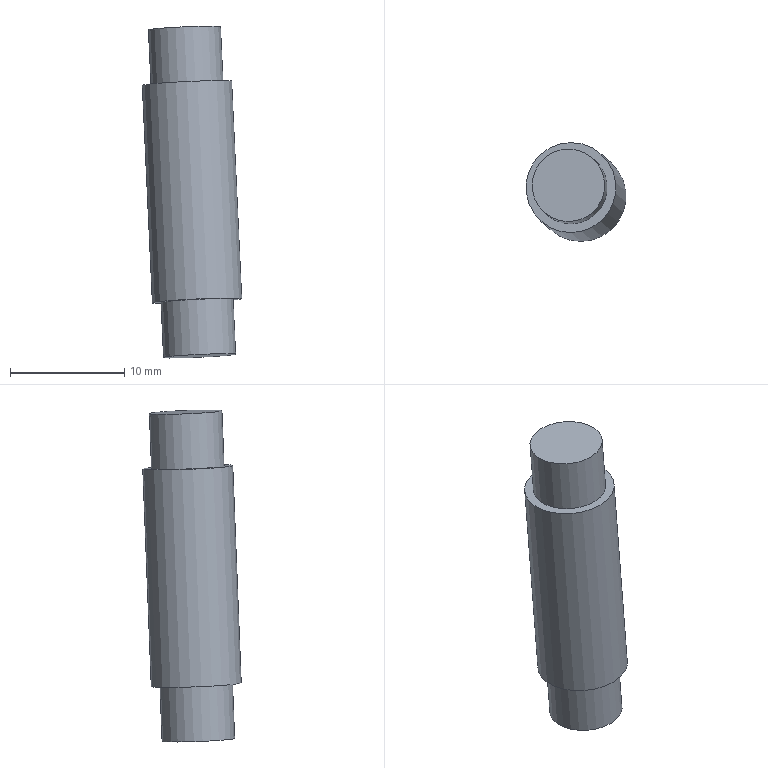Component | NX | PASADOR_A_2 | 1 solid | 7 faces | box 8.75 x 8.61 x 29.03 mm | volume 1233 mm3 | plane 4 | cylinder 3 | commonest cylinder face diameters 6.35 x2 7.874 x1
STEP:
#1=CARTESIAN_POINT('',(0.,0.,0.));
#2=DIRECTION('',(0.,0.,1.));
#3=DIRECTION('',(1.,0.,0.));
#4=AXIS2_PLACEMENT_3D('',#1,#2,#3);
#5=CARTESIAN_POINT('',(4.095,61.023,10.643));
#6=VERTEX_POINT('',#5);
#7=CARTESIAN_POINT('',(0.1942,61.516,10.443));
#8=DIRECTION('',(-0.04625,0.03881,0.9982));
#9=DIRECTION('',(0.9908,-0.1251,0.05077));
#10=AXIS2_PLACEMENT_3D('',#7,#8,#9);
#11=CIRCLE('',#10,3.937);
#12=CARTESIAN_POINT('',(0.1942,61.516,10.443));
#13=DIRECTION('',(-0.04625,0.03881,0.9982));
#14=DIRECTION('',(0.9908,-0.1251,0.05077));
#15=AXIS2_PLACEMENT_3D('',#12,#13,#14);
#16=PLANE('',#15);
#17=CARTESIAN_POINT('',(0.,0.));
#18=DIRECTION('',(1.,-0.));
#19=AXIS2_PLACEMENT_2D('',#17,#18);
#20=CIRCLE('',#19,3.937);
#21=(GEOMETRIC_REPRESENTATION_CONTEXT(2)PARAMETRIC_REPRESENTATION_CONTEXT()REPRESENTATION_CONTEXT('',''));
#22=DEFINITIONAL_REPRESENTATION('',(#20),#21);
#23=PCURVE('',#16,#22);
#24=CARTESIAN_POINT('',(0.1942,61.516,10.443));
#25=DIRECTION('',(0.04625,-0.03881,-0.9982));
#26=DIRECTION('',(-0.9908,0.1251,-0.05077));
#27=AXIS2_PLACEMENT_3D('',#24,#25,#26);
#28=CYLINDRICAL_SURFACE('',#27,3.937);
#29=CARTESIAN_POINT('',(9.425,0.));
#30=DIRECTION('',(-1.,0.));
#31=VECTOR('',#30,1.);
#32=LINE('',#29,#31);
#33=(GEOMETRIC_REPRESENTATION_CONTEXT(2)PARAMETRIC_REPRESENTATION_CONTEXT()REPRESENTATION_CONTEXT('',''));
#34=DEFINITIONAL_REPRESENTATION('',(#32),#33);
#35=PCURVE('',#28,#34);
#36=SURFACE_CURVE('',#11,(#23,#35),.PCURVE_S1.);
#37=EDGE_CURVE('',#6,#6,#36,.T.);
#38=ORIENTED_EDGE('',*,*,#37,.T.);
#39=EDGE_LOOP('',(#38));
#40=FACE_BOUND('',#39,.T.);
#41=CARTESIAN_POINT('',(3.34,61.119,10.604));
#42=VERTEX_POINT('',#41);
#43=CARTESIAN_POINT('',(0.1942,61.516,10.443));
#44=DIRECTION('',(0.04625,-0.03881,-0.9982));
#45=DIRECTION('',(0.9908,-0.1251,0.05077));
#46=AXIS2_PLACEMENT_3D('',#43,#44,#45);
#47=CIRCLE('',#46,3.175);
#48=CARTESIAN_POINT('',(3.175,-0.));
#49=CARTESIAN_POINT('',(3.175,-5.499));
#50=CARTESIAN_POINT('',(-1.587,-2.75));
#51=CARTESIAN_POINT('',(-6.35,0.));
#52=CARTESIAN_POINT('',(-1.587,2.75));
#53=CARTESIAN_POINT('',(3.175,5.499));
#54=CARTESIAN_POINT('',(3.175,-0.));
#55=(BOUNDED_CURVE()B_SPLINE_CURVE(2,(#48,#49,#50,#51,#52,#53,#54),.UNSPECIFIED.,.T.,.F.)B_SPLINE_CURVE_WITH_KNOTS((1,2,2,2,2,1),(-2.094,0.,2.094,4.189,6.283,8.378),.UNSPECIFIED.)CURVE()GEOMETRIC_REPRESENTATION_ITEM()RATIONAL_B_SPLINE_CURVE((1.,0.5,1.,0.5,1.,0.5,1.))REPRESENTATION_ITEM(''));
#56=(GEOMETRIC_REPRESENTATION_CONTEXT(2)PARAMETRIC_REPRESENTATION_CONTEXT()REPRESENTATION_CONTEXT('',''));
#57=DEFINITIONAL_REPRESENTATION('',(#55),#56);
#58=PCURVE('',#16,#57);
#59=CARTESIAN_POINT('',(-0.02899,61.703,15.26));
#60=DIRECTION('',(0.04625,-0.03881,-0.9982));
#61=DIRECTION('',(-0.9908,0.1251,-0.05077));
#62=AXIS2_PLACEMENT_3D('',#59,#60,#61);
#63=CYLINDRICAL_SURFACE('',#62,3.175);
#64=CARTESIAN_POINT('',(3.142,4.826));
#65=DIRECTION('',(1.,0.));
#66=VECTOR('',#65,1.);
#67=LINE('',#64,#66);
#68=(GEOMETRIC_REPRESENTATION_CONTEXT(2)PARAMETRIC_REPRESENTATION_CONTEXT()REPRESENTATION_CONTEXT('',''));
#69=DEFINITIONAL_REPRESENTATION('',(#67),#68);
#70=PCURVE('',#63,#69);
#71=SURFACE_CURVE('',#47,(#58,#70),.PCURVE_S1.);
#72=EDGE_CURVE('',#42,#42,#71,.T.);
#73=ORIENTED_EDGE('',*,*,#72,.T.);
#74=EDGE_LOOP('',(#73));
#75=FACE_BOUND('',#74,.T.);
#76=ADVANCED_FACE('',(#40,#75),#16,.T.);
#77=CARTESIAN_POINT('',(4.976,60.284,-8.372));
#78=VERTEX_POINT('',#77);
#79=CARTESIAN_POINT('',(1.075,60.777,-8.572));
#80=DIRECTION('',(-0.04625,0.03881,0.9982));
#81=DIRECTION('',(0.9908,-0.1251,0.05077));
#82=AXIS2_PLACEMENT_3D('',#79,#80,#81);
#83=CIRCLE('',#82,3.937);
#84=CARTESIAN_POINT('',(1.075,60.777,-8.572));
#85=DIRECTION('',(-0.04625,0.03881,0.9982));
#86=DIRECTION('',(0.9908,-0.1251,0.05077));
#87=AXIS2_PLACEMENT_3D('',#84,#85,#86);
#88=PLANE('',#87);
#89=CARTESIAN_POINT('',(0.,0.));
#90=DIRECTION('',(1.,-0.));
#91=AXIS2_PLACEMENT_2D('',#89,#90);
#92=CIRCLE('',#91,3.937);
#93=(GEOMETRIC_REPRESENTATION_CONTEXT(2)PARAMETRIC_REPRESENTATION_CONTEXT()REPRESENTATION_CONTEXT('',''));
#94=DEFINITIONAL_REPRESENTATION('',(#92),#93);
#95=PCURVE('',#88,#94);
#96=CARTESIAN_POINT('',(9.425,19.05));
#97=DIRECTION('',(-1.,0.));
#98=VECTOR('',#97,1.);
#99=LINE('',#96,#98);
#100=(GEOMETRIC_REPRESENTATION_CONTEXT(2)PARAMETRIC_REPRESENTATION_CONTEXT()REPRESENTATION_CONTEXT('',''));
#101=DEFINITIONAL_REPRESENTATION('',(#99),#100);
#102=PCURVE('',#28,#101);
#103=SURFACE_CURVE('',#83,(#95,#102),.PCURVE_S1.);
#104=EDGE_CURVE('',#78,#78,#103,.T.);
#105=ORIENTED_EDGE('',*,*,#104,.F.);
#106=EDGE_LOOP('',(#105));
#107=FACE_BOUND('',#106,.T.);
#108=CARTESIAN_POINT('',(4.221,60.38,-8.411));
#109=VERTEX_POINT('',#108);
#110=CARTESIAN_POINT('',(1.075,60.777,-8.572));
#111=DIRECTION('',(0.04625,-0.03881,-0.9982));
#112=DIRECTION('',(0.9908,-0.1251,0.05077));
#113=AXIS2_PLACEMENT_3D('',#110,#111,#112);
#114=CIRCLE('',#113,3.175);
#115=CARTESIAN_POINT('',(3.175,-0.));
#116=CARTESIAN_POINT('',(3.175,-5.499));
#117=CARTESIAN_POINT('',(-1.587,-2.75));
#118=CARTESIAN_POINT('',(-6.35,0.));
#119=CARTESIAN_POINT('',(-1.587,2.75));
#120=CARTESIAN_POINT('',(3.175,5.499));
#121=CARTESIAN_POINT('',(3.175,-0.));
#122=(BOUNDED_CURVE()B_SPLINE_CURVE(2,(#115,#116,#117,#118,#119,#120,#121),.UNSPECIFIED.,.T.,.F.)B_SPLINE_CURVE_WITH_KNOTS((1,2,2,2,2,1),(-2.094,0.,2.094,4.189,6.283,8.378),.UNSPECIFIED.)CURVE()GEOMETRIC_REPRESENTATION_ITEM()RATIONAL_B_SPLINE_CURVE((1.,0.5,1.,0.5,1.,0.5,1.))REPRESENTATION_ITEM(''));
#123=(GEOMETRIC_REPRESENTATION_CONTEXT(2)PARAMETRIC_REPRESENTATION_CONTEXT()REPRESENTATION_CONTEXT('',''));
#124=DEFINITIONAL_REPRESENTATION('',(#122),#123);
#125=PCURVE('',#88,#124);
#126=CARTESIAN_POINT('',(-0.02899,61.703,15.26));
#127=DIRECTION('',(0.04625,-0.03881,-0.9982));
#128=DIRECTION('',(-0.9908,0.1251,-0.05077));
#129=AXIS2_PLACEMENT_3D('',#126,#127,#128);
#130=CYLINDRICAL_SURFACE('',#129,3.175);
#131=CARTESIAN_POINT('',(3.142,23.876));
#132=DIRECTION('',(1.,0.));
#133=VECTOR('',#132,1.);
#134=LINE('',#131,#133);
#135=(GEOMETRIC_REPRESENTATION_CONTEXT(2)PARAMETRIC_REPRESENTATION_CONTEXT()REPRESENTATION_CONTEXT('',''));
#136=DEFINITIONAL_REPRESENTATION('',(#134),#135);
#137=PCURVE('',#130,#136);
#138=SURFACE_CURVE('',#114,(#125,#137),.PCURVE_S1.);
#139=EDGE_CURVE('',#109,#109,#138,.T.);
#140=ORIENTED_EDGE('',*,*,#139,.F.);
#141=EDGE_LOOP('',(#140));
#142=FACE_BOUND('',#141,.T.);
#143=ADVANCED_FACE('',(#107,#142),#88,.F.);
#144=ORIENTED_EDGE('',*,*,#37,.F.);
#145=CARTESIAN_POINT('',(4.095,61.023,10.643));
#146=CARTESIAN_POINT('',(4.976,60.284,-8.372));
#147=B_SPLINE_CURVE_WITH_KNOTS('',1,(#145,#146),.UNSPECIFIED.,.F.,.F.,(2,2),(0.,19.05),.PIECEWISE_BEZIER_KNOTS.);
#148=CARTESIAN_POINT('',(9.425,0.));
#149=DIRECTION('',(0.,1.));
#150=VECTOR('',#149,1.);
#151=LINE('',#148,#150);
#152=(GEOMETRIC_REPRESENTATION_CONTEXT(2)PARAMETRIC_REPRESENTATION_CONTEXT()REPRESENTATION_CONTEXT('',''));
#153=DEFINITIONAL_REPRESENTATION('',(#151),#152);
#154=PCURVE('',#28,#153);
#155=CARTESIAN_POINT('',(3.142,0.));
#156=DIRECTION('',(0.,1.));
#157=VECTOR('',#156,1.);
#158=LINE('',#155,#157);
#159=(GEOMETRIC_REPRESENTATION_CONTEXT(2)PARAMETRIC_REPRESENTATION_CONTEXT()REPRESENTATION_CONTEXT('',''));
#160=DEFINITIONAL_REPRESENTATION('',(#158),#159);
#161=PCURVE('',#28,#160);
#162=SEAM_CURVE('',#147,(#154,#161),.PCURVE_S1.);
#163=EDGE_CURVE('',#6,#78,#162,.T.);
#164=ORIENTED_EDGE('',*,*,#163,.T.);
#165=ORIENTED_EDGE('',*,*,#104,.T.);
#166=ORIENTED_EDGE('',*,*,#163,.F.);
#167=EDGE_LOOP('',(#144,#164,#165,#166));
#168=FACE_BOUND('',#167,.T.);
#169=ADVANCED_FACE('',(#168),#28,.T.);
#170=CARTESIAN_POINT('',(4.444,60.192,-13.228));
#171=VERTEX_POINT('',#170);
#172=CARTESIAN_POINT('',(1.298,60.589,-13.389));
#173=DIRECTION('',(-0.04625,0.03881,0.9982));
#174=DIRECTION('',(0.9908,-0.1251,0.05077));
#175=AXIS2_PLACEMENT_3D('',#172,#173,#174);
#176=CIRCLE('',#175,3.175);
#177=CARTESIAN_POINT('',(1.298,60.589,-13.389));
#178=DIRECTION('',(-0.04625,0.03881,0.9982));
#179=DIRECTION('',(0.9908,-0.1251,0.05077));
#180=AXIS2_PLACEMENT_3D('',#177,#178,#179);
#181=PLANE('',#180);
#182=CARTESIAN_POINT('',(0.,0.));
#183=DIRECTION('',(1.,-0.));
#184=AXIS2_PLACEMENT_2D('',#182,#183);
#185=CIRCLE('',#184,3.175);
#186=(GEOMETRIC_REPRESENTATION_CONTEXT(2)PARAMETRIC_REPRESENTATION_CONTEXT()REPRESENTATION_CONTEXT('',''));
#187=DEFINITIONAL_REPRESENTATION('',(#185),#186);
#188=PCURVE('',#181,#187);
#189=CARTESIAN_POINT('',(9.425,28.702));
#190=DIRECTION('',(-1.,0.));
#191=VECTOR('',#190,1.);
#192=LINE('',#189,#191);
#193=(GEOMETRIC_REPRESENTATION_CONTEXT(2)PARAMETRIC_REPRESENTATION_CONTEXT()REPRESENTATION_CONTEXT('',''));
#194=DEFINITIONAL_REPRESENTATION('',(#192),#193);
#195=PCURVE('',#130,#194);
#196=SURFACE_CURVE('',#176,(#188,#195),.PCURVE_S1.);
#197=EDGE_CURVE('',#171,#171,#196,.T.);
#198=ORIENTED_EDGE('',*,*,#197,.F.);
#199=EDGE_LOOP('',(#198));
#200=FACE_BOUND('',#199,.T.);
#201=ADVANCED_FACE('',(#200),#181,.F.);
#202=ORIENTED_EDGE('',*,*,#197,.T.);
#203=CARTESIAN_POINT('',(4.221,60.38,-8.411));
#204=CARTESIAN_POINT('',(4.444,60.192,-13.228));
#205=B_SPLINE_CURVE_WITH_KNOTS('',1,(#203,#204),.UNSPECIFIED.,.F.,.F.,(2,2),(23.876,28.702),.PIECEWISE_BEZIER_KNOTS.);
#206=CARTESIAN_POINT('',(3.142,0.));
#207=DIRECTION('',(0.,1.));
#208=VECTOR('',#207,1.);
#209=LINE('',#206,#208);
#210=(GEOMETRIC_REPRESENTATION_CONTEXT(2)PARAMETRIC_REPRESENTATION_CONTEXT()REPRESENTATION_CONTEXT('',''));
#211=DEFINITIONAL_REPRESENTATION('',(#209),#210);
#212=PCURVE('',#130,#211);
#213=CARTESIAN_POINT('',(9.425,0.));
#214=DIRECTION('',(0.,1.));
#215=VECTOR('',#214,1.);
#216=LINE('',#213,#215);
#217=(GEOMETRIC_REPRESENTATION_CONTEXT(2)PARAMETRIC_REPRESENTATION_CONTEXT()REPRESENTATION_CONTEXT('',''));
#218=DEFINITIONAL_REPRESENTATION('',(#216),#217);
#219=PCURVE('',#130,#218);
#220=SEAM_CURVE('',#205,(#212,#219),.PCURVE_S1.);
#221=EDGE_CURVE('',#109,#171,#220,.T.);
#222=ORIENTED_EDGE('',*,*,#221,.F.);
#223=ORIENTED_EDGE('',*,*,#139,.T.);
#224=ORIENTED_EDGE('',*,*,#221,.T.);
#225=EDGE_LOOP('',(#202,#222,#223,#224));
#226=FACE_BOUND('',#225,.T.);
#227=ADVANCED_FACE('',(#226),#130,.T.);
#228=ORIENTED_EDGE('',*,*,#72,.F.);
#229=CARTESIAN_POINT('',(3.117,61.306,15.421));
#230=VERTEX_POINT('',#229);
#231=CARTESIAN_POINT('',(3.117,61.306,15.421));
#232=CARTESIAN_POINT('',(3.34,61.119,10.604));
#233=B_SPLINE_CURVE_WITH_KNOTS('',1,(#231,#232),.UNSPECIFIED.,.F.,.F.,(2,2),(-0.,4.826),.PIECEWISE_BEZIER_KNOTS.);
#234=CARTESIAN_POINT('',(3.142,0.));
#235=DIRECTION('',(0.,1.));
#236=VECTOR('',#235,1.);
#237=LINE('',#234,#236);
#238=(GEOMETRIC_REPRESENTATION_CONTEXT(2)PARAMETRIC_REPRESENTATION_CONTEXT()REPRESENTATION_CONTEXT('',''));
#239=DEFINITIONAL_REPRESENTATION('',(#237),#238);
#240=PCURVE('',#63,#239);
#241=CARTESIAN_POINT('',(9.425,0.));
#242=DIRECTION('',(0.,1.));
#243=VECTOR('',#242,1.);
#244=LINE('',#241,#243);
#245=(GEOMETRIC_REPRESENTATION_CONTEXT(2)PARAMETRIC_REPRESENTATION_CONTEXT()REPRESENTATION_CONTEXT('',''));
#246=DEFINITIONAL_REPRESENTATION('',(#244),#245);
#247=PCURVE('',#63,#246);
#248=SEAM_CURVE('',#233,(#240,#247),.PCURVE_S1.);
#249=EDGE_CURVE('',#230,#42,#248,.T.);
#250=ORIENTED_EDGE('',*,*,#249,.F.);
#251=CARTESIAN_POINT('',(-0.02899,61.703,15.26));
#252=DIRECTION('',(-0.04625,0.03881,0.9982));
#253=DIRECTION('',(0.9908,-0.1251,0.05077));
#254=AXIS2_PLACEMENT_3D('',#251,#252,#253);
#255=CIRCLE('',#254,3.175);
#256=CARTESIAN_POINT('',(9.425,-0.));
#257=DIRECTION('',(-1.,0.));
#258=VECTOR('',#257,1.);
#259=LINE('',#256,#258);
#260=(GEOMETRIC_REPRESENTATION_CONTEXT(2)PARAMETRIC_REPRESENTATION_CONTEXT()REPRESENTATION_CONTEXT('',''));
#261=DEFINITIONAL_REPRESENTATION('',(#259),#260);
#262=PCURVE('',#63,#261);
#263=CARTESIAN_POINT('',(-0.02899,61.703,15.26));
#264=DIRECTION('',(-0.04625,0.03881,0.9982));
#265=DIRECTION('',(0.9908,-0.1251,0.05077));
#266=AXIS2_PLACEMENT_3D('',#263,#264,#265);
#267=PLANE('',#266);
#268=CARTESIAN_POINT('',(0.,0.));
#269=DIRECTION('',(1.,-0.));
#270=AXIS2_PLACEMENT_2D('',#268,#269);
#271=CIRCLE('',#270,3.175);
#272=(GEOMETRIC_REPRESENTATION_CONTEXT(2)PARAMETRIC_REPRESENTATION_CONTEXT()REPRESENTATION_CONTEXT('',''));
#273=DEFINITIONAL_REPRESENTATION('',(#271),#272);
#274=PCURVE('',#267,#273);
#275=SURFACE_CURVE('',#255,(#262,#274),.PCURVE_S1.);
#276=EDGE_CURVE('',#230,#230,#275,.T.);
#277=ORIENTED_EDGE('',*,*,#276,.F.);
#278=ORIENTED_EDGE('',*,*,#249,.T.);
#279=EDGE_LOOP('',(#228,#250,#277,#278));
#280=FACE_BOUND('',#279,.T.);
#281=ADVANCED_FACE('',(#280),#63,.T.);
#282=ORIENTED_EDGE('',*,*,#276,.T.);
#283=EDGE_LOOP('',(#282));
#284=FACE_BOUND('',#283,.T.);
#285=ADVANCED_FACE('',(#284),#267,.T.);
#286=CLOSED_SHELL('',(#76,#143,#169,#201,#227,#281,#285));
#287=MANIFOLD_SOLID_BREP('',#286);
#288=(LENGTH_UNIT()NAMED_UNIT(*)SI_UNIT(.MILLI.,.METRE.));
#289=UNCERTAINTY_MEASURE_WITH_UNIT(LENGTH_MEASURE(0.00001),#288,'','');
#290=(NAMED_UNIT(*)PLANE_ANGLE_UNIT()SI_UNIT($,.RADIAN.));
#291=(NAMED_UNIT(*)SI_UNIT($,.STERADIAN.)SOLID_ANGLE_UNIT());
#292=(GEOMETRIC_REPRESENTATION_CONTEXT(3)GLOBAL_UNCERTAINTY_ASSIGNED_CONTEXT((#289))GLOBAL_UNIT_ASSIGNED_CONTEXT((#288,#290,#291))REPRESENTATION_CONTEXT('',''));
#293=ADVANCED_BREP_SHAPE_REPRESENTATION('',(#4,#287),#292);